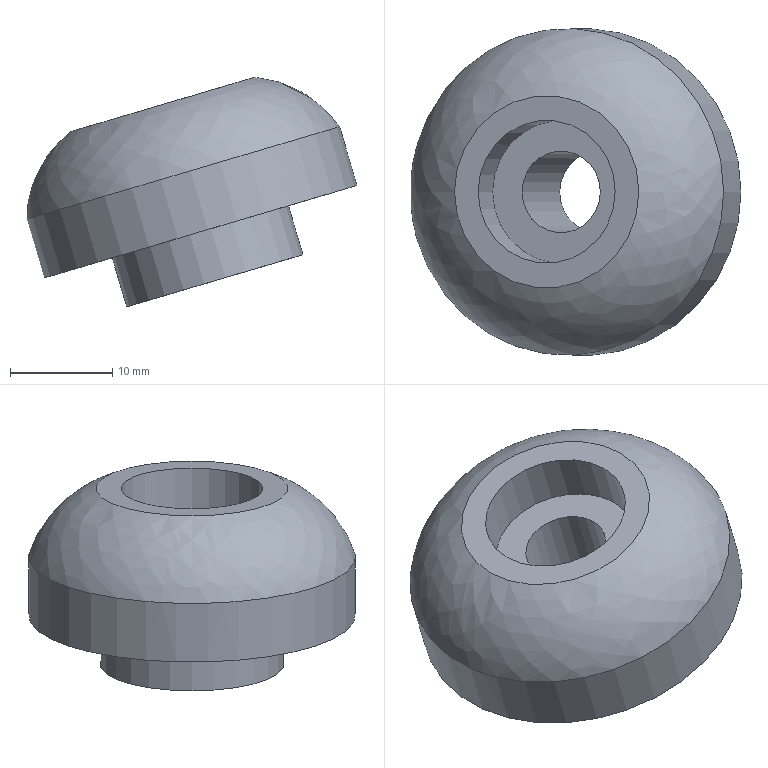Component | NX | HANDLE | 1 solid | 9 faces | box 32.39 x 32 x 22.48 mm | volume 8871 mm3 | plane 4 | cylinder 4 | spline 1 | commonest cylinder face diameters 18 x1 32 x1 8 x1 14 x1
STEP:
#1=CARTESIAN_POINT('',(0.,0.,0.));
#2=DIRECTION('',(0.,0.,1.));
#3=DIRECTION('',(1.,0.,0.));
#4=AXIS2_PLACEMENT_3D('',#1,#2,#3);
#5=CARTESIAN_POINT('',(102.997,0.,151.521));
#6=VERTEX_POINT('',#5);
#7=CARTESIAN_POINT('',(106.832,0.,152.655));
#8=DIRECTION('',(-0.2835,0.,0.959));
#9=DIRECTION('',(-0.959,0.,-0.2835));
#10=AXIS2_PLACEMENT_3D('',#7,#8,#9);
#11=CIRCLE('',#10,4.);
#12=CARTESIAN_POINT('',(106.832,-9.,152.655));
#13=DIRECTION('',(0.2835,0.,-0.959));
#14=DIRECTION('',(-0.959,0.,-0.2835));
#15=AXIS2_PLACEMENT_3D('',#12,#13,#14);
#16=PLANE('',#15);
#17=CARTESIAN_POINT('',(4.,9.));
#18=CARTESIAN_POINT('',(4.,2.072));
#19=CARTESIAN_POINT('',(-2.,5.536));
#20=CARTESIAN_POINT('',(-8.,9.));
#21=CARTESIAN_POINT('',(-2.,12.464));
#22=CARTESIAN_POINT('',(4.,15.928));
#23=CARTESIAN_POINT('',(4.,9.));
#24=(BOUNDED_CURVE()B_SPLINE_CURVE(2,(#17,#18,#19,#20,#21,#22,#23),.UNSPECIFIED.,.T.,.F.)B_SPLINE_CURVE_WITH_KNOTS((1,2,2,2,2,1),(-2.094,0.,2.094,4.189,6.283,8.378),.UNSPECIFIED.)CURVE()GEOMETRIC_REPRESENTATION_ITEM()RATIONAL_B_SPLINE_CURVE((1.,0.5,1.,0.5,1.,0.5,1.))REPRESENTATION_ITEM(''));
#25=(GEOMETRIC_REPRESENTATION_CONTEXT(2)PARAMETRIC_REPRESENTATION_CONTEXT()REPRESENTATION_CONTEXT('',''));
#26=DEFINITIONAL_REPRESENTATION('',(#24),#25);
#27=PCURVE('',#16,#26);
#28=CARTESIAN_POINT('',(110.519,0.,140.189));
#29=DIRECTION('',(-0.2835,0.,0.959));
#30=DIRECTION('',(0.959,0.,0.2835));
#31=AXIS2_PLACEMENT_3D('',#28,#29,#30);
#32=CYLINDRICAL_SURFACE('',#31,4.);
#33=CARTESIAN_POINT('',(3.142,13.));
#34=DIRECTION('',(1.,0.));
#35=VECTOR('',#34,1.);
#36=LINE('',#33,#35);
#37=(GEOMETRIC_REPRESENTATION_CONTEXT(2)PARAMETRIC_REPRESENTATION_CONTEXT()REPRESENTATION_CONTEXT('',''));
#38=DEFINITIONAL_REPRESENTATION('',(#36),#37);
#39=PCURVE('',#32,#38);
#40=SURFACE_CURVE('',#11,(#27,#39),.PCURVE_S1.);
#41=EDGE_CURVE('',#6,#6,#40,.T.);
#42=ORIENTED_EDGE('',*,*,#41,.T.);
#43=EDGE_LOOP('',(#42));
#44=FACE_BOUND('',#43,.T.);
#45=CARTESIAN_POINT('',(115.463,0.,155.207));
#46=VERTEX_POINT('',#45);
#47=CARTESIAN_POINT('',(106.832,0.,152.655));
#48=DIRECTION('',(-0.2835,0.,0.959));
#49=DIRECTION('',(0.959,0.,0.2835));
#50=AXIS2_PLACEMENT_3D('',#47,#48,#49);
#51=CIRCLE('',#50,9.);
#52=CARTESIAN_POINT('',(-9.,9.));
#53=CARTESIAN_POINT('',(-9.,24.588));
#54=CARTESIAN_POINT('',(4.5,16.794));
#55=CARTESIAN_POINT('',(18.,9.));
#56=CARTESIAN_POINT('',(4.5,1.206));
#57=CARTESIAN_POINT('',(-9.,-6.588));
#58=CARTESIAN_POINT('',(-9.,9.));
#59=(BOUNDED_CURVE()B_SPLINE_CURVE(2,(#52,#53,#54,#55,#56,#57,#58),.UNSPECIFIED.,.T.,.F.)B_SPLINE_CURVE_WITH_KNOTS((1,2,2,2,2,1),(-2.094,0.,2.094,4.189,6.283,8.378),.UNSPECIFIED.)CURVE()GEOMETRIC_REPRESENTATION_ITEM()RATIONAL_B_SPLINE_CURVE((1.,0.5,1.,0.5,1.,0.5,1.))REPRESENTATION_ITEM(''));
#60=(GEOMETRIC_REPRESENTATION_CONTEXT(2)PARAMETRIC_REPRESENTATION_CONTEXT()REPRESENTATION_CONTEXT('',''));
#61=DEFINITIONAL_REPRESENTATION('',(#59),#60);
#62=PCURVE('',#16,#61);
#63=CARTESIAN_POINT('',(106.832,0.,152.655));
#64=DIRECTION('',(-0.2835,0.,0.959));
#65=DIRECTION('',(0.959,0.,0.2835));
#66=AXIS2_PLACEMENT_3D('',#63,#64,#65);
#67=CYLINDRICAL_SURFACE('',#66,9.);
#68=CARTESIAN_POINT('',(0.,-0.));
#69=DIRECTION('',(1.,0.));
#70=VECTOR('',#69,1.);
#71=LINE('',#68,#70);
#72=(GEOMETRIC_REPRESENTATION_CONTEXT(2)PARAMETRIC_REPRESENTATION_CONTEXT()REPRESENTATION_CONTEXT('',''));
#73=DEFINITIONAL_REPRESENTATION('',(#71),#72);
#74=PCURVE('',#67,#73);
#75=SURFACE_CURVE('',#51,(#62,#74),.PCURVE_S1.);
#76=EDGE_CURVE('',#46,#46,#75,.T.);
#77=ORIENTED_EDGE('',*,*,#76,.F.);
#78=EDGE_LOOP('',(#77));
#79=FACE_BOUND('',#78,.T.);
#80=ADVANCED_FACE('',(#44,#79),#16,.T.);
#81=ORIENTED_EDGE('',*,*,#76,.T.);
#82=CARTESIAN_POINT('',(114.045,0.,160.002));
#83=VERTEX_POINT('',#82);
#84=CARTESIAN_POINT('',(115.463,0.,155.207));
#85=CARTESIAN_POINT('',(114.045,0.,160.002));
#86=B_SPLINE_CURVE_WITH_KNOTS('',1,(#84,#85),.UNSPECIFIED.,.F.,.F.,(2,2),(-0.,5.),.PIECEWISE_BEZIER_KNOTS.);
#87=CARTESIAN_POINT('',(6.283,0.));
#88=DIRECTION('',(0.,1.));
#89=VECTOR('',#88,1.);
#90=LINE('',#87,#89);
#91=(GEOMETRIC_REPRESENTATION_CONTEXT(2)PARAMETRIC_REPRESENTATION_CONTEXT()REPRESENTATION_CONTEXT('',''));
#92=DEFINITIONAL_REPRESENTATION('',(#90),#91);
#93=PCURVE('',#67,#92);
#94=CARTESIAN_POINT('',(0.,0.));
#95=DIRECTION('',(0.,1.));
#96=VECTOR('',#95,1.);
#97=LINE('',#94,#96);
#98=(GEOMETRIC_REPRESENTATION_CONTEXT(2)PARAMETRIC_REPRESENTATION_CONTEXT()REPRESENTATION_CONTEXT('',''));
#99=DEFINITIONAL_REPRESENTATION('',(#97),#98);
#100=PCURVE('',#67,#99);
#101=SEAM_CURVE('',#86,(#93,#100),.PCURVE_S1.);
#102=EDGE_CURVE('',#46,#83,#101,.T.);
#103=ORIENTED_EDGE('',*,*,#102,.T.);
#104=CARTESIAN_POINT('',(105.415,0.,157.45));
#105=DIRECTION('',(-0.2835,0.,0.959));
#106=DIRECTION('',(0.959,0.,0.2835));
#107=AXIS2_PLACEMENT_3D('',#104,#105,#106);
#108=CIRCLE('',#107,9.);
#109=CARTESIAN_POINT('',(0.,5.));
#110=DIRECTION('',(1.,0.));
#111=VECTOR('',#110,1.);
#112=LINE('',#109,#111);
#113=(GEOMETRIC_REPRESENTATION_CONTEXT(2)PARAMETRIC_REPRESENTATION_CONTEXT()REPRESENTATION_CONTEXT('',''));
#114=DEFINITIONAL_REPRESENTATION('',(#112),#113);
#115=PCURVE('',#67,#114);
#116=CARTESIAN_POINT('',(105.415,-16.,157.45));
#117=DIRECTION('',(0.2835,0.,-0.959));
#118=DIRECTION('',(-0.959,0.,-0.2835));
#119=AXIS2_PLACEMENT_3D('',#116,#117,#118);
#120=PLANE('',#119);
#121=CARTESIAN_POINT('',(-9.,16.));
#122=CARTESIAN_POINT('',(-9.,31.588));
#123=CARTESIAN_POINT('',(4.5,23.794));
#124=CARTESIAN_POINT('',(18.,16.));
#125=CARTESIAN_POINT('',(4.5,8.206));
#126=CARTESIAN_POINT('',(-9.,0.4115));
#127=CARTESIAN_POINT('',(-9.,16.));
#128=(BOUNDED_CURVE()B_SPLINE_CURVE(2,(#121,#122,#123,#124,#125,#126,#127),.UNSPECIFIED.,.T.,.F.)B_SPLINE_CURVE_WITH_KNOTS((1,2,2,2,2,1),(-2.094,0.,2.094,4.189,6.283,8.378),.UNSPECIFIED.)CURVE()GEOMETRIC_REPRESENTATION_ITEM()RATIONAL_B_SPLINE_CURVE((1.,0.5,1.,0.5,1.,0.5,1.))REPRESENTATION_ITEM(''));
#129=(GEOMETRIC_REPRESENTATION_CONTEXT(2)PARAMETRIC_REPRESENTATION_CONTEXT()REPRESENTATION_CONTEXT('',''));
#130=DEFINITIONAL_REPRESENTATION('',(#128),#129);
#131=PCURVE('',#120,#130);
#132=SURFACE_CURVE('',#108,(#115,#131),.PCURVE_S1.);
#133=EDGE_CURVE('',#83,#83,#132,.T.);
#134=ORIENTED_EDGE('',*,*,#133,.F.);
#135=ORIENTED_EDGE('',*,*,#102,.F.);
#136=EDGE_LOOP('',(#81,#103,#134,#135));
#137=FACE_BOUND('',#136,.T.);
#138=ADVANCED_FACE('',(#137),#67,.T.);
#139=ORIENTED_EDGE('',*,*,#133,.T.);
#140=EDGE_LOOP('',(#139));
#141=FACE_BOUND('',#140,.T.);
#142=CARTESIAN_POINT('',(120.758,0.,161.987));
#143=VERTEX_POINT('',#142);
#144=CARTESIAN_POINT('',(105.415,0.,157.45));
#145=DIRECTION('',(-0.2835,0.,0.959));
#146=DIRECTION('',(0.959,0.,0.2835));
#147=AXIS2_PLACEMENT_3D('',#144,#145,#146);
#148=CIRCLE('',#147,16.);
#149=CARTESIAN_POINT('',(-16.,16.));
#150=CARTESIAN_POINT('',(-16.,43.713));
#151=CARTESIAN_POINT('',(8.,29.856));
#152=CARTESIAN_POINT('',(32.,16.));
#153=CARTESIAN_POINT('',(8.,2.144));
#154=CARTESIAN_POINT('',(-16.,-11.713));
#155=CARTESIAN_POINT('',(-16.,16.));
#156=(BOUNDED_CURVE()B_SPLINE_CURVE(2,(#149,#150,#151,#152,#153,#154,#155),.UNSPECIFIED.,.T.,.F.)B_SPLINE_CURVE_WITH_KNOTS((1,2,2,2,2,1),(-2.094,0.,2.094,4.189,6.283,8.378),.UNSPECIFIED.)CURVE()GEOMETRIC_REPRESENTATION_ITEM()RATIONAL_B_SPLINE_CURVE((1.,0.5,1.,0.5,1.,0.5,1.))REPRESENTATION_ITEM(''));
#157=(GEOMETRIC_REPRESENTATION_CONTEXT(2)PARAMETRIC_REPRESENTATION_CONTEXT()REPRESENTATION_CONTEXT('',''));
#158=DEFINITIONAL_REPRESENTATION('',(#156),#157);
#159=PCURVE('',#120,#158);
#160=CARTESIAN_POINT('',(106.832,0.,152.655));
#161=DIRECTION('',(-0.2835,0.,0.959));
#162=DIRECTION('',(0.959,0.,0.2835));
#163=AXIS2_PLACEMENT_3D('',#160,#161,#162);
#164=CYLINDRICAL_SURFACE('',#163,16.);
#165=CARTESIAN_POINT('',(0.,5.));
#166=DIRECTION('',(1.,0.));
#167=VECTOR('',#166,1.);
#168=LINE('',#165,#167);
#169=(GEOMETRIC_REPRESENTATION_CONTEXT(2)PARAMETRIC_REPRESENTATION_CONTEXT()REPRESENTATION_CONTEXT('',''));
#170=DEFINITIONAL_REPRESENTATION('',(#168),#169);
#171=PCURVE('',#164,#170);
#172=SURFACE_CURVE('',#148,(#159,#171),.PCURVE_S1.);
#173=EDGE_CURVE('',#143,#143,#172,.T.);
#174=ORIENTED_EDGE('',*,*,#173,.F.);
#175=EDGE_LOOP('',(#174));
#176=FACE_BOUND('',#175,.T.);
#177=ADVANCED_FACE('',(#141,#176),#120,.T.);
#178=ORIENTED_EDGE('',*,*,#173,.T.);
#179=CARTESIAN_POINT('',(119.057,0.,167.741));
#180=VERTEX_POINT('',#179);
#181=CARTESIAN_POINT('',(120.758,0.,161.987));
#182=CARTESIAN_POINT('',(119.057,0.,167.741));
#183=B_SPLINE_CURVE_WITH_KNOTS('',1,(#181,#182),.UNSPECIFIED.,.F.,.F.,(2,2),(5.,11.),.PIECEWISE_BEZIER_KNOTS.);
#184=CARTESIAN_POINT('',(6.283,0.));
#185=DIRECTION('',(0.,1.));
#186=VECTOR('',#185,1.);
#187=LINE('',#184,#186);
#188=(GEOMETRIC_REPRESENTATION_CONTEXT(2)PARAMETRIC_REPRESENTATION_CONTEXT()REPRESENTATION_CONTEXT('',''));
#189=DEFINITIONAL_REPRESENTATION('',(#187),#188);
#190=PCURVE('',#164,#189);
#191=CARTESIAN_POINT('',(0.,0.));
#192=DIRECTION('',(0.,1.));
#193=VECTOR('',#192,1.);
#194=LINE('',#191,#193);
#195=(GEOMETRIC_REPRESENTATION_CONTEXT(2)PARAMETRIC_REPRESENTATION_CONTEXT()REPRESENTATION_CONTEXT('',''));
#196=DEFINITIONAL_REPRESENTATION('',(#194),#195);
#197=PCURVE('',#164,#196);
#198=SEAM_CURVE('',#183,(#190,#197),.PCURVE_S1.);
#199=EDGE_CURVE('',#143,#180,#198,.T.);
#200=ORIENTED_EDGE('',*,*,#199,.T.);
#201=CARTESIAN_POINT('',(103.713,0.,163.204));
#202=DIRECTION('',(-0.2835,0.,0.959));
#203=DIRECTION('',(0.959,0.,0.2835));
#204=AXIS2_PLACEMENT_3D('',#201,#202,#203);
#205=CIRCLE('',#204,16.);
#206=CARTESIAN_POINT('',(0.,11.));
#207=DIRECTION('',(1.,0.));
#208=VECTOR('',#207,1.);
#209=LINE('',#206,#208);
#210=(GEOMETRIC_REPRESENTATION_CONTEXT(2)PARAMETRIC_REPRESENTATION_CONTEXT()REPRESENTATION_CONTEXT('',''));
#211=DEFINITIONAL_REPRESENTATION('',(#209),#210);
#212=PCURVE('',#164,#211);
#213=CARTESIAN_POINT('',(110.762,0.,172.588));
#214=CARTESIAN_POINT('',(110.762,18.84,172.588));
#215=CARTESIAN_POINT('',(92.695,18.84,167.246));
#216=CARTESIAN_POINT('',(92.695,0.,167.246));
#217=CARTESIAN_POINT('',(92.695,-18.84,167.246));
#218=CARTESIAN_POINT('',(110.762,-18.84,172.588));
#219=CARTESIAN_POINT('',(110.762,0.,172.588));
#220=CARTESIAN_POINT('',(114.167,0.,172.282));
#221=CARTESIAN_POINT('',(114.167,25.197,172.282));
#222=CARTESIAN_POINT('',(90.004,25.197,165.137));
#223=CARTESIAN_POINT('',(90.004,0.,165.137));
#224=CARTESIAN_POINT('',(90.004,-25.197,165.137));
#225=CARTESIAN_POINT('',(114.167,-25.197,172.282));
#226=CARTESIAN_POINT('',(114.167,0.,172.282));
#227=CARTESIAN_POINT('',(117.119,0.,170.557));
#228=CARTESIAN_POINT('',(117.119,29.88,170.557));
#229=CARTESIAN_POINT('',(88.465,29.88,162.085));
#230=CARTESIAN_POINT('',(88.465,0.,162.085));
#231=CARTESIAN_POINT('',(88.465,-29.88,162.085));
#232=CARTESIAN_POINT('',(117.119,-29.88,170.557));
#233=CARTESIAN_POINT('',(117.119,0.,170.557));
#234=CARTESIAN_POINT('',(119.057,0.,167.741));
#235=CARTESIAN_POINT('',(119.057,32.,167.741));
#236=CARTESIAN_POINT('',(88.37,32.,158.667));
#237=CARTESIAN_POINT('',(88.37,0.,158.667));
#238=CARTESIAN_POINT('',(88.37,-32.,158.667));
#239=CARTESIAN_POINT('',(119.057,-32.,167.741));
#240=CARTESIAN_POINT('',(119.057,0.,167.741));
#241=(BOUNDED_SURFACE()B_SPLINE_SURFACE(3,3,((#213,#214,#215,#216,#217,#218,#219),(#220,#221,#222,#223,#224,#225,#226),(#227,#228,#229,#230,#231,#232,#233),(#234,#235,#236,#237,#238,#239,#240)),.UNSPECIFIED.,.F.,.T.,.F.)B_SPLINE_SURFACE_WITH_KNOTS((4,4),(1,3,3,3,1),(0.,1.),(-0.5,0.,0.5,1.,1.5),.UNSPECIFIED.)GEOMETRIC_REPRESENTATION_ITEM()RATIONAL_B_SPLINE_SURFACE(((1.,0.3333,0.3333,1.,0.3333,0.3333,1.),(0.9367,0.3122,0.3122,0.9367,0.3122,0.3122,0.9367),(0.9367,0.3122,0.3122,0.9367,0.3122,0.3122,0.9367),(1.,0.3333,0.3333,1.,0.3333,0.3333,1.)))REPRESENTATION_ITEM('')SURFACE());
#242=CARTESIAN_POINT('',(1.,0.));
#243=CARTESIAN_POINT('',(1.,0.02352));
#244=CARTESIAN_POINT('',(1.,0.06491));
#245=CARTESIAN_POINT('',(1.,0.1146));
#246=CARTESIAN_POINT('',(1.,0.1575));
#247=CARTESIAN_POINT('',(1.,0.196));
#248=CARTESIAN_POINT('',(1.,0.2322));
#249=CARTESIAN_POINT('',(1.,0.2678));
#250=CARTESIAN_POINT('',(1.,0.304));
#251=CARTESIAN_POINT('',(1.,0.3425));
#252=CARTESIAN_POINT('',(1.,0.3856));
#253=CARTESIAN_POINT('',(1.,0.4343));
#254=CARTESIAN_POINT('',(1.,0.5));
#255=CARTESIAN_POINT('',(1.,0.5657));
#256=CARTESIAN_POINT('',(1.,0.6144));
#257=CARTESIAN_POINT('',(1.,0.6575));
#258=CARTESIAN_POINT('',(1.,0.696));
#259=CARTESIAN_POINT('',(1.,0.7322));
#260=CARTESIAN_POINT('',(1.,0.7678));
#261=CARTESIAN_POINT('',(1.,0.804));
#262=CARTESIAN_POINT('',(1.,0.8425));
#263=CARTESIAN_POINT('',(1.,0.8854));
#264=CARTESIAN_POINT('',(1.,0.9351));
#265=CARTESIAN_POINT('',(1.,0.9765));
#266=CARTESIAN_POINT('',(1.,1.));
#267=B_SPLINE_CURVE_WITH_KNOTS('',3,(#242,#243,#244,#245,#246,#247,#248,#249,#250,#251,#252,#253,#254,#255,#256,#257,#258,#259,#260,#261,#262,#263,#264,#265,#266),.UNSPECIFIED.,.F.,.F.,(4,1,1,1,1,1,1,1,1,1,1,1,1,1,1,1,1,1,1,1,1,1,4),(0.,0.2856,0.5712,0.8568,1.142,1.428,1.714,1.999,2.285,2.57,2.856,3.142,3.427,3.713,3.998,4.284,4.57,4.855,5.141,5.426,5.712,5.998,6.283),.QUASI_UNIFORM_KNOTS.);
#268=(GEOMETRIC_REPRESENTATION_CONTEXT(2)PARAMETRIC_REPRESENTATION_CONTEXT()REPRESENTATION_CONTEXT('',''));
#269=DEFINITIONAL_REPRESENTATION('',(#267),#268);
#270=PCURVE('',#241,#269);
#271=SURFACE_CURVE('',#205,(#212,#270),.PCURVE_S1.);
#272=EDGE_CURVE('',#180,#180,#271,.T.);
#273=ORIENTED_EDGE('',*,*,#272,.F.);
#274=ORIENTED_EDGE('',*,*,#199,.F.);
#275=EDGE_LOOP('',(#178,#200,#273,#274));
#276=FACE_BOUND('',#275,.T.);
#277=ADVANCED_FACE('',(#276),#164,.T.);
#278=ORIENTED_EDGE('',*,*,#272,.T.);
#279=CARTESIAN_POINT('',(110.762,0.,172.588));
#280=VERTEX_POINT('',#279);
#281=CARTESIAN_POINT('',(110.762,0.,172.588));
#282=CARTESIAN_POINT('',(114.167,0.,172.282));
#283=CARTESIAN_POINT('',(117.119,0.,170.557));
#284=CARTESIAN_POINT('',(119.057,0.,167.741));
#285=(BOUNDED_CURVE()B_SPLINE_CURVE(3,(#281,#282,#283,#284),.UNSPECIFIED.,.F.,.F.)B_SPLINE_CURVE_WITH_KNOTS((4,4),(0.,1.),.PIECEWISE_BEZIER_KNOTS.)CURVE()GEOMETRIC_REPRESENTATION_ITEM()RATIONAL_B_SPLINE_CURVE((1.,0.9367,0.9367,1.))REPRESENTATION_ITEM(''));
#286=CARTESIAN_POINT('',(0.,1.));
#287=DIRECTION('',(1.,0.));
#288=VECTOR('',#287,1.);
#289=LINE('',#286,#288);
#290=(GEOMETRIC_REPRESENTATION_CONTEXT(2)PARAMETRIC_REPRESENTATION_CONTEXT()REPRESENTATION_CONTEXT('',''));
#291=DEFINITIONAL_REPRESENTATION('',(#289),#290);
#292=PCURVE('',#241,#291);
#293=CARTESIAN_POINT('',(0.,0.));
#294=DIRECTION('',(1.,0.));
#295=VECTOR('',#294,1.);
#296=LINE('',#293,#295);
#297=(GEOMETRIC_REPRESENTATION_CONTEXT(2)PARAMETRIC_REPRESENTATION_CONTEXT()REPRESENTATION_CONTEXT('',''));
#298=DEFINITIONAL_REPRESENTATION('',(#296),#297);
#299=PCURVE('',#241,#298);
#300=SEAM_CURVE('',#285,(#292,#299),.PCURVE_S1.);
#301=EDGE_CURVE('',#280,#180,#300,.T.);
#302=ORIENTED_EDGE('',*,*,#301,.F.);
#303=CARTESIAN_POINT('',(101.729,0.,169.917));
#304=DIRECTION('',(-0.2835,0.,0.959));
#305=DIRECTION('',(0.959,0.,0.2835));
#306=AXIS2_PLACEMENT_3D('',#303,#304,#305);
#307=CIRCLE('',#306,9.42);
#308=CARTESIAN_POINT('',(0.,0.));
#309=CARTESIAN_POINT('',(0.,0.02352));
#310=CARTESIAN_POINT('',(0.,0.06491));
#311=CARTESIAN_POINT('',(0.,0.1146));
#312=CARTESIAN_POINT('',(0.,0.1575));
#313=CARTESIAN_POINT('',(0.,0.196));
#314=CARTESIAN_POINT('',(0.,0.2322));
#315=CARTESIAN_POINT('',(0.,0.2678));
#316=CARTESIAN_POINT('',(0.,0.304));
#317=CARTESIAN_POINT('',(0.,0.3425));
#318=CARTESIAN_POINT('',(0.,0.3856));
#319=CARTESIAN_POINT('',(0.,0.4343));
#320=CARTESIAN_POINT('',(0.,0.5));
#321=CARTESIAN_POINT('',(0.,0.5657));
#322=CARTESIAN_POINT('',(0.,0.6144));
#323=CARTESIAN_POINT('',(0.,0.6575));
#324=CARTESIAN_POINT('',(0.,0.696));
#325=CARTESIAN_POINT('',(0.,0.7322));
#326=CARTESIAN_POINT('',(0.,0.7678));
#327=CARTESIAN_POINT('',(0.,0.804));
#328=CARTESIAN_POINT('',(0.,0.8425));
#329=CARTESIAN_POINT('',(0.,0.8854));
#330=CARTESIAN_POINT('',(0.,0.9351));
#331=CARTESIAN_POINT('',(0.,0.9765));
#332=CARTESIAN_POINT('',(0.,1.));
#333=B_SPLINE_CURVE_WITH_KNOTS('',3,(#308,#309,#310,#311,#312,#313,#314,#315,#316,#317,#318,#319,#320,#321,#322,#323,#324,#325,#326,#327,#328,#329,#330,#331,#332),.UNSPECIFIED.,.F.,.F.,(4,1,1,1,1,1,1,1,1,1,1,1,1,1,1,1,1,1,1,1,1,1,4),(0.,0.2856,0.5712,0.8568,1.142,1.428,1.714,1.999,2.285,2.57,2.856,3.142,3.427,3.713,3.998,4.284,4.57,4.855,5.141,5.426,5.712,5.998,6.283),.QUASI_UNIFORM_KNOTS.);
#334=(GEOMETRIC_REPRESENTATION_CONTEXT(2)PARAMETRIC_REPRESENTATION_CONTEXT()REPRESENTATION_CONTEXT('',''));
#335=DEFINITIONAL_REPRESENTATION('',(#333),#334);
#336=PCURVE('',#241,#335);
#337=CARTESIAN_POINT('',(101.729,0.,169.917));
#338=DIRECTION('',(-0.2835,0.,0.959));
#339=DIRECTION('',(0.959,0.,0.2835));
#340=AXIS2_PLACEMENT_3D('',#337,#338,#339);
#341=PLANE('',#340);
#342=CARTESIAN_POINT('',(0.,0.));
#343=DIRECTION('',(1.,0.));
#344=AXIS2_PLACEMENT_2D('',#342,#343);
#345=CIRCLE('',#344,9.42);
#346=(GEOMETRIC_REPRESENTATION_CONTEXT(2)PARAMETRIC_REPRESENTATION_CONTEXT()REPRESENTATION_CONTEXT('',''));
#347=DEFINITIONAL_REPRESENTATION('',(#345),#346);
#348=PCURVE('',#341,#347);
#349=SURFACE_CURVE('',#307,(#336,#348),.PCURVE_S1.);
#350=EDGE_CURVE('',#280,#280,#349,.T.);
#351=ORIENTED_EDGE('',*,*,#350,.F.);
#352=ORIENTED_EDGE('',*,*,#301,.T.);
#353=EDGE_LOOP('',(#278,#302,#351,#352));
#354=FACE_BOUND('',#353,.T.);
#355=ADVANCED_FACE('',(#354),#241,.T.);
#356=CARTESIAN_POINT('',(108.441,0.,171.902));
#357=VERTEX_POINT('',#356);
#358=CARTESIAN_POINT('',(101.729,0.,169.917));
#359=DIRECTION('',(0.2835,0.,-0.959));
#360=DIRECTION('',(0.959,0.,0.2835));
#361=AXIS2_PLACEMENT_3D('',#358,#359,#360);
#362=CIRCLE('',#361,7.);
#363=CARTESIAN_POINT('',(7.,0.));
#364=CARTESIAN_POINT('',(7.,-12.124));
#365=CARTESIAN_POINT('',(-3.5,-6.062));
#366=CARTESIAN_POINT('',(-14.,-0.));
#367=CARTESIAN_POINT('',(-3.5,6.062));
#368=CARTESIAN_POINT('',(7.,12.124));
#369=CARTESIAN_POINT('',(7.,0.));
#370=(BOUNDED_CURVE()B_SPLINE_CURVE(2,(#363,#364,#365,#366,#367,#368,#369),.UNSPECIFIED.,.T.,.F.)B_SPLINE_CURVE_WITH_KNOTS((1,2,2,2,2,1),(-2.094,0.,2.094,4.189,6.283,8.378),.UNSPECIFIED.)CURVE()GEOMETRIC_REPRESENTATION_ITEM()RATIONAL_B_SPLINE_CURVE((1.,0.5,1.,0.5,1.,0.5,1.))REPRESENTATION_ITEM(''));
#371=(GEOMETRIC_REPRESENTATION_CONTEXT(2)PARAMETRIC_REPRESENTATION_CONTEXT()REPRESENTATION_CONTEXT('',''));
#372=DEFINITIONAL_REPRESENTATION('',(#370),#371);
#373=PCURVE('',#341,#372);
#374=CARTESIAN_POINT('',(103.146,0.,165.122));
#375=DIRECTION('',(-0.2835,0.,0.959));
#376=DIRECTION('',(0.959,0.,0.2835));
#377=AXIS2_PLACEMENT_3D('',#374,#375,#376);
#378=CYLINDRICAL_SURFACE('',#377,7.);
#379=CARTESIAN_POINT('',(6.283,5.));
#380=DIRECTION('',(-1.,0.));
#381=VECTOR('',#380,1.);
#382=LINE('',#379,#381);
#383=(GEOMETRIC_REPRESENTATION_CONTEXT(2)PARAMETRIC_REPRESENTATION_CONTEXT()REPRESENTATION_CONTEXT('',''));
#384=DEFINITIONAL_REPRESENTATION('',(#382),#383);
#385=PCURVE('',#378,#384);
#386=SURFACE_CURVE('',#362,(#373,#385),.PCURVE_S1.);
#387=EDGE_CURVE('',#357,#357,#386,.T.);
#388=ORIENTED_EDGE('',*,*,#387,.T.);
#389=EDGE_LOOP('',(#388));
#390=FACE_BOUND('',#389,.T.);
#391=ORIENTED_EDGE('',*,*,#350,.T.);
#392=EDGE_LOOP('',(#391));
#393=FACE_BOUND('',#392,.T.);
#394=ADVANCED_FACE('',(#390,#393),#341,.T.);
#395=CARTESIAN_POINT('',(99.311,0.,163.988));
#396=VERTEX_POINT('',#395);
#397=CARTESIAN_POINT('',(103.146,0.,165.122));
#398=DIRECTION('',(0.2835,0.,-0.959));
#399=DIRECTION('',(-0.959,0.,-0.2835));
#400=AXIS2_PLACEMENT_3D('',#397,#398,#399);
#401=CIRCLE('',#400,4.);
#402=CARTESIAN_POINT('',(9.425,26.));
#403=DIRECTION('',(-1.,0.));
#404=VECTOR('',#403,1.);
#405=LINE('',#402,#404);
#406=(GEOMETRIC_REPRESENTATION_CONTEXT(2)PARAMETRIC_REPRESENTATION_CONTEXT()REPRESENTATION_CONTEXT('',''));
#407=DEFINITIONAL_REPRESENTATION('',(#405),#406);
#408=PCURVE('',#32,#407);
#409=CARTESIAN_POINT('',(103.146,0.,165.122));
#410=DIRECTION('',(0.2835,0.,-0.959));
#411=DIRECTION('',(-0.959,0.,-0.2835));
#412=AXIS2_PLACEMENT_3D('',#409,#410,#411);
#413=PLANE('',#412);
#414=CARTESIAN_POINT('',(0.,0.));
#415=DIRECTION('',(1.,0.));
#416=AXIS2_PLACEMENT_2D('',#414,#415);
#417=CIRCLE('',#416,4.);
#418=(GEOMETRIC_REPRESENTATION_CONTEXT(2)PARAMETRIC_REPRESENTATION_CONTEXT()REPRESENTATION_CONTEXT('',''));
#419=DEFINITIONAL_REPRESENTATION('',(#417),#418);
#420=PCURVE('',#413,#419);
#421=SURFACE_CURVE('',#401,(#408,#420),.PCURVE_S1.);
#422=EDGE_CURVE('',#396,#396,#421,.T.);
#423=ORIENTED_EDGE('',*,*,#422,.T.);
#424=CARTESIAN_POINT('',(102.997,0.,151.521));
#425=CARTESIAN_POINT('',(99.311,0.,163.988));
#426=B_SPLINE_CURVE_WITH_KNOTS('',1,(#424,#425),.UNSPECIFIED.,.F.,.F.,(2,2),(13.,26.),.PIECEWISE_BEZIER_KNOTS.);
#427=CARTESIAN_POINT('',(3.142,0.));
#428=DIRECTION('',(0.,1.));
#429=VECTOR('',#428,1.);
#430=LINE('',#427,#429);
#431=(GEOMETRIC_REPRESENTATION_CONTEXT(2)PARAMETRIC_REPRESENTATION_CONTEXT()REPRESENTATION_CONTEXT('',''));
#432=DEFINITIONAL_REPRESENTATION('',(#430),#431);
#433=PCURVE('',#32,#432);
#434=CARTESIAN_POINT('',(9.425,0.));
#435=DIRECTION('',(0.,1.));
#436=VECTOR('',#435,1.);
#437=LINE('',#434,#436);
#438=(GEOMETRIC_REPRESENTATION_CONTEXT(2)PARAMETRIC_REPRESENTATION_CONTEXT()REPRESENTATION_CONTEXT('',''));
#439=DEFINITIONAL_REPRESENTATION('',(#437),#438);
#440=PCURVE('',#32,#439);
#441=SEAM_CURVE('',#426,(#433,#440),.PCURVE_S1.);
#442=EDGE_CURVE('',#6,#396,#441,.T.);
#443=ORIENTED_EDGE('',*,*,#442,.F.);
#444=ORIENTED_EDGE('',*,*,#41,.T.);
#445=ORIENTED_EDGE('',*,*,#442,.T.);
#446=EDGE_LOOP('',(#423,#443,#444,#445));
#447=FACE_BOUND('',#446,.F.);
#448=ADVANCED_FACE('',(#447),#32,.F.);
#449=CARTESIAN_POINT('',(109.859,0.,167.107));
#450=VERTEX_POINT('',#449);
#451=CARTESIAN_POINT('',(103.146,0.,165.122));
#452=DIRECTION('',(-0.2835,0.,0.959));
#453=DIRECTION('',(0.959,0.,0.2835));
#454=AXIS2_PLACEMENT_3D('',#451,#452,#453);
#455=CIRCLE('',#454,7.);
#456=CARTESIAN_POINT('',(0.,0.));
#457=DIRECTION('',(1.,0.));
#458=VECTOR('',#457,1.);
#459=LINE('',#456,#458);
#460=(GEOMETRIC_REPRESENTATION_CONTEXT(2)PARAMETRIC_REPRESENTATION_CONTEXT()REPRESENTATION_CONTEXT('',''));
#461=DEFINITIONAL_REPRESENTATION('',(#459),#460);
#462=PCURVE('',#378,#461);
#463=CARTESIAN_POINT('',(-7.,0.));
#464=CARTESIAN_POINT('',(-7.,12.124));
#465=CARTESIAN_POINT('',(3.5,6.062));
#466=CARTESIAN_POINT('',(14.,0.));
#467=CARTESIAN_POINT('',(3.5,-6.062));
#468=CARTESIAN_POINT('',(-7.,-12.124));
#469=CARTESIAN_POINT('',(-7.,0.));
#470=(BOUNDED_CURVE()B_SPLINE_CURVE(2,(#463,#464,#465,#466,#467,#468,#469),.UNSPECIFIED.,.T.,.F.)B_SPLINE_CURVE_WITH_KNOTS((1,2,2,2,2,1),(-2.094,0.,2.094,4.189,6.283,8.378),.UNSPECIFIED.)CURVE()GEOMETRIC_REPRESENTATION_ITEM()RATIONAL_B_SPLINE_CURVE((1.,0.5,1.,0.5,1.,0.5,1.))REPRESENTATION_ITEM(''));
#471=(GEOMETRIC_REPRESENTATION_CONTEXT(2)PARAMETRIC_REPRESENTATION_CONTEXT()REPRESENTATION_CONTEXT('',''));
#472=DEFINITIONAL_REPRESENTATION('',(#470),#471);
#473=PCURVE('',#413,#472);
#474=SURFACE_CURVE('',#455,(#462,#473),.PCURVE_S1.);
#475=EDGE_CURVE('',#450,#450,#474,.T.);
#476=ORIENTED_EDGE('',*,*,#475,.T.);
#477=CARTESIAN_POINT('',(109.859,0.,167.107));
#478=CARTESIAN_POINT('',(108.441,0.,171.902));
#479=B_SPLINE_CURVE_WITH_KNOTS('',1,(#477,#478),.UNSPECIFIED.,.F.,.F.,(2,2),(0.,5.),.PIECEWISE_BEZIER_KNOTS.);
#480=CARTESIAN_POINT('',(6.283,0.));
#481=DIRECTION('',(0.,1.));
#482=VECTOR('',#481,1.);
#483=LINE('',#480,#482);
#484=(GEOMETRIC_REPRESENTATION_CONTEXT(2)PARAMETRIC_REPRESENTATION_CONTEXT()REPRESENTATION_CONTEXT('',''));
#485=DEFINITIONAL_REPRESENTATION('',(#483),#484);
#486=PCURVE('',#378,#485);
#487=CARTESIAN_POINT('',(0.,0.));
#488=DIRECTION('',(0.,1.));
#489=VECTOR('',#488,1.);
#490=LINE('',#487,#489);
#491=(GEOMETRIC_REPRESENTATION_CONTEXT(2)PARAMETRIC_REPRESENTATION_CONTEXT()REPRESENTATION_CONTEXT('',''));
#492=DEFINITIONAL_REPRESENTATION('',(#490),#491);
#493=PCURVE('',#378,#492);
#494=SEAM_CURVE('',#479,(#486,#493),.PCURVE_S1.);
#495=EDGE_CURVE('',#450,#357,#494,.T.);
#496=ORIENTED_EDGE('',*,*,#495,.T.);
#497=ORIENTED_EDGE('',*,*,#387,.T.);
#498=ORIENTED_EDGE('',*,*,#495,.F.);
#499=EDGE_LOOP('',(#476,#496,#497,#498));
#500=FACE_BOUND('',#499,.F.);
#501=ADVANCED_FACE('',(#500),#378,.F.);
#502=ORIENTED_EDGE('',*,*,#422,.T.);
#503=EDGE_LOOP('',(#502));
#504=FACE_BOUND('',#503,.T.);
#505=ORIENTED_EDGE('',*,*,#475,.T.);
#506=EDGE_LOOP('',(#505));
#507=FACE_BOUND('',#506,.T.);
#508=ADVANCED_FACE('',(#504,#507),#413,.F.);
#509=CLOSED_SHELL('',(#80,#138,#177,#277,#355,#394,#448,#501,#508));
#510=MANIFOLD_SOLID_BREP('',#509);
#511=(LENGTH_UNIT()NAMED_UNIT(*)SI_UNIT(.MILLI.,.METRE.));
#512=UNCERTAINTY_MEASURE_WITH_UNIT(LENGTH_MEASURE(0.00001),#511,'','');
#513=(NAMED_UNIT(*)PLANE_ANGLE_UNIT()SI_UNIT($,.RADIAN.));
#514=(NAMED_UNIT(*)SI_UNIT($,.STERADIAN.)SOLID_ANGLE_UNIT());
#515=(GEOMETRIC_REPRESENTATION_CONTEXT(3)GLOBAL_UNCERTAINTY_ASSIGNED_CONTEXT((#512))GLOBAL_UNIT_ASSIGNED_CONTEXT((#511,#513,#514))REPRESENTATION_CONTEXT('',''));
#516=ADVANCED_BREP_SHAPE_REPRESENTATION('',(#4,#510),#515);